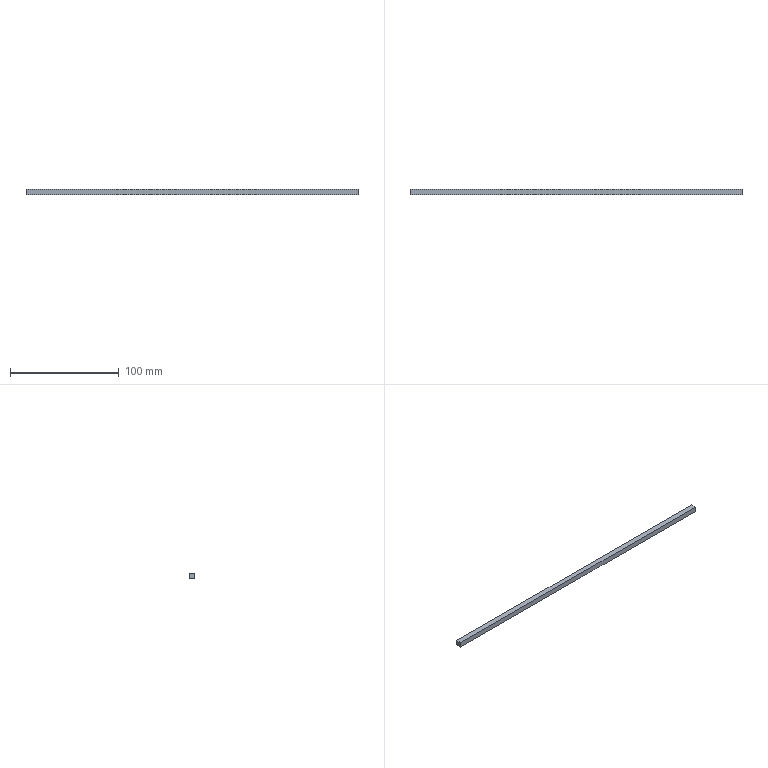Component | SolidWorks | Part23-1 | 1 solid | 6 faces | box 305.58 x 5 x 4.86 mm | volume 7420 mm3 | plane 6
build123d program:
from build123d import *

# Parameters (mm, degrees)
SKETCH1_W           = 4.857
SKETCH1_H           = 5
BOSS_EXTRUDE1_DEPTH = 305.58


with BuildPart() as part:
    # Sketch1 → Boss-Extrude1 (new body)
    with BuildSketch(Plane.XY):
        with Locations((276.879, 308.428)):
            Rectangle(SKETCH1_W, SKETCH1_H)
    extrude(amount=-BOSS_EXTRUDE1_DEPTH)


solid = part.part

# Placed as in the assembly
solid = solid.moved(Location((152.794, -25.683, -135.592), (0, 90, 0)))
STEP:
#1=CARTESIAN_POINT('',(6.016,11.23,-16.143));
#2=VERTEX_POINT('',#1);
#3=CARTESIAN_POINT('',(6.016,11.033,-16.143));
#4=VERTEX_POINT('',#3);
#5=CARTESIAN_POINT('',(6.016,11.23,-16.143));
#6=DIRECTION('',(0.,-1.,0.));
#7=VECTOR('',#6,39.37);
#8=LINE('',#5,#7);
#9=EDGE_CURVE('',#2,#4,#8,.T.);
#10=ORIENTED_EDGE('',*,*,#9,.F.);
#11=CARTESIAN_POINT('',(-6.015,11.23,-16.143));
#12=VERTEX_POINT('',#11);
#13=CARTESIAN_POINT('',(-6.015,11.23,-16.143));
#14=DIRECTION('',(1.,0.,0.));
#15=VECTOR('',#14,39.37);
#16=LINE('',#13,#15);
#17=EDGE_CURVE('',#12,#2,#16,.T.);
#18=ORIENTED_EDGE('',*,*,#17,.F.);
#19=CARTESIAN_POINT('',(-6.015,11.033,-16.143));
#20=VERTEX_POINT('',#19);
#21=CARTESIAN_POINT('',(-6.015,11.23,-16.143));
#22=DIRECTION('',(0.,-1.,0.));
#23=VECTOR('',#22,39.37);
#24=LINE('',#21,#23);
#25=EDGE_CURVE('',#12,#20,#24,.T.);
#26=ORIENTED_EDGE('',*,*,#25,.T.);
#27=CARTESIAN_POINT('',(-6.015,11.033,-16.143));
#28=DIRECTION('',(1.,0.,0.));
#29=VECTOR('',#28,39.37);
#30=LINE('',#27,#29);
#31=EDGE_CURVE('',#20,#4,#30,.T.);
#32=ORIENTED_EDGE('',*,*,#31,.T.);
#33=EDGE_LOOP('',(#10,#18,#26,#32));
#34=FACE_OUTER_BOUND('',#33,.T.);
#35=CARTESIAN_POINT('',(-6.015,11.23,-16.143));
#36=DIRECTION('',(0.,0.,1.));
#37=DIRECTION('',(1.,0.,0.));
#38=AXIS2_PLACEMENT_3D('',#35,#36,#37);
#39=PLANE('',#38);
#40=ADVANCED_FACE('',(#34),#39,.T.);
#41=CARTESIAN_POINT('',(6.016,11.23,-16.335));
#42=VERTEX_POINT('',#41);
#43=CARTESIAN_POINT('',(6.016,11.23,-16.143));
#44=DIRECTION('',(0.,0.,1.));
#45=VECTOR('',#44,39.37);
#46=LINE('',#43,#45);
#47=EDGE_CURVE('',#42,#2,#46,.T.);
#48=ORIENTED_EDGE('',*,*,#47,.F.);
#49=CARTESIAN_POINT('',(-6.015,11.23,-16.335));
#50=VERTEX_POINT('',#49);
#51=CARTESIAN_POINT('',(-6.015,11.23,-16.335));
#52=DIRECTION('',(1.,0.,0.));
#53=VECTOR('',#52,39.37);
#54=LINE('',#51,#53);
#55=EDGE_CURVE('',#50,#42,#54,.T.);
#56=ORIENTED_EDGE('',*,*,#55,.F.);
#57=CARTESIAN_POINT('',(-6.015,11.23,-16.143));
#58=DIRECTION('',(0.,0.,1.));
#59=VECTOR('',#58,39.37);
#60=LINE('',#57,#59);
#61=EDGE_CURVE('',#50,#12,#60,.T.);
#62=ORIENTED_EDGE('',*,*,#61,.T.);
#63=ORIENTED_EDGE('',*,*,#17,.T.);
#64=EDGE_LOOP('',(#48,#56,#62,#63));
#65=FACE_OUTER_BOUND('',#64,.T.);
#66=CARTESIAN_POINT('',(-6.015,11.23,-16.143));
#67=DIRECTION('',(0.,1.,0.));
#68=DIRECTION('',(1.,0.,0.));
#69=AXIS2_PLACEMENT_3D('',#66,#67,#68);
#70=PLANE('',#69);
#71=ADVANCED_FACE('',(#65),#70,.T.);
#72=CARTESIAN_POINT('',(6.016,11.033,-16.335));
#73=VERTEX_POINT('',#72);
#74=CARTESIAN_POINT('',(6.016,11.23,-16.335));
#75=DIRECTION('',(0.,1.,0.));
#76=VECTOR('',#75,39.37);
#77=LINE('',#74,#76);
#78=EDGE_CURVE('',#73,#42,#77,.T.);
#79=ORIENTED_EDGE('',*,*,#78,.F.);
#80=CARTESIAN_POINT('',(-6.015,11.033,-16.335));
#81=VERTEX_POINT('',#80);
#82=CARTESIAN_POINT('',(-6.015,11.033,-16.335));
#83=DIRECTION('',(1.,0.,0.));
#84=VECTOR('',#83,39.37);
#85=LINE('',#82,#84);
#86=EDGE_CURVE('',#81,#73,#85,.T.);
#87=ORIENTED_EDGE('',*,*,#86,.F.);
#88=CARTESIAN_POINT('',(-6.015,11.23,-16.335));
#89=DIRECTION('',(0.,1.,0.));
#90=VECTOR('',#89,39.37);
#91=LINE('',#88,#90);
#92=EDGE_CURVE('',#81,#50,#91,.T.);
#93=ORIENTED_EDGE('',*,*,#92,.T.);
#94=ORIENTED_EDGE('',*,*,#55,.T.);
#95=EDGE_LOOP('',(#79,#87,#93,#94));
#96=FACE_OUTER_BOUND('',#95,.T.);
#97=CARTESIAN_POINT('',(-6.015,11.23,-16.335));
#98=DIRECTION('',(0.,0.,-1.));
#99=DIRECTION('',(-1.,0.,0.));
#100=AXIS2_PLACEMENT_3D('',#97,#98,#99);
#101=PLANE('',#100);
#102=ADVANCED_FACE('',(#96),#101,.T.);
#103=CARTESIAN_POINT('',(6.016,11.033,-16.143));
#104=DIRECTION('',(0.,0.,-1.));
#105=VECTOR('',#104,39.37);
#106=LINE('',#103,#105);
#107=EDGE_CURVE('',#4,#73,#106,.T.);
#108=ORIENTED_EDGE('',*,*,#107,.F.);
#109=ORIENTED_EDGE('',*,*,#31,.F.);
#110=CARTESIAN_POINT('',(-6.015,11.033,-16.143));
#111=DIRECTION('',(0.,0.,-1.));
#112=VECTOR('',#111,39.37);
#113=LINE('',#110,#112);
#114=EDGE_CURVE('',#20,#81,#113,.T.);
#115=ORIENTED_EDGE('',*,*,#114,.T.);
#116=ORIENTED_EDGE('',*,*,#86,.T.);
#117=EDGE_LOOP('',(#108,#109,#115,#116));
#118=FACE_OUTER_BOUND('',#117,.T.);
#119=CARTESIAN_POINT('',(-6.015,11.033,-16.143));
#120=DIRECTION('',(0.,-1.,0.));
#121=DIRECTION('',(-1.,0.,0.));
#122=AXIS2_PLACEMENT_3D('',#119,#120,#121);
#123=PLANE('',#122);
#124=ADVANCED_FACE('',(#118),#123,.T.);
#125=ORIENTED_EDGE('',*,*,#25,.F.);
#126=ORIENTED_EDGE('',*,*,#61,.F.);
#127=ORIENTED_EDGE('',*,*,#92,.F.);
#128=ORIENTED_EDGE('',*,*,#114,.F.);
#129=EDGE_LOOP('',(#125,#126,#127,#128));
#130=FACE_OUTER_BOUND('',#129,.T.);
#131=CARTESIAN_POINT('',(-6.015,-1.011,-5.338));
#132=DIRECTION('',(1.,0.,0.));
#133=DIRECTION('',(0.,0.,-1.));
#134=AXIS2_PLACEMENT_3D('',#131,#132,#133);
#135=PLANE('',#134);
#136=ADVANCED_FACE('',(#130),#135,.F.);
#137=ORIENTED_EDGE('',*,*,#9,.T.);
#138=ORIENTED_EDGE('',*,*,#107,.T.);
#139=ORIENTED_EDGE('',*,*,#78,.T.);
#140=ORIENTED_EDGE('',*,*,#47,.T.);
#141=EDGE_LOOP('',(#137,#138,#139,#140));
#142=FACE_OUTER_BOUND('',#141,.T.);
#143=CARTESIAN_POINT('',(6.016,-1.011,-5.338));
#144=DIRECTION('',(1.,0.,0.));
#145=DIRECTION('',(0.,0.,-1.));
#146=AXIS2_PLACEMENT_3D('',#143,#144,#145);
#147=PLANE('',#146);
#148=ADVANCED_FACE('',(#142),#147,.T.);
#149=CLOSED_SHELL('',(#40,#71,#102,#124,#136,#148));
#150=MANIFOLD_SOLID_BREP('',#149);
#151=CARTESIAN_POINT('',(0.,0.,0.));
#152=DIRECTION('',(0.,0.,1.));
#153=DIRECTION('',(1.,0.,0.));
#154=AXIS2_PLACEMENT_3D('',#151,#152,#153);
#155=(LENGTH_UNIT()NAMED_UNIT(*)SI_UNIT($,.METRE.));
#156=LENGTH_MEASURE_WITH_UNIT(LENGTH_MEASURE(0.0254),#155);
#157=DIMENSIONAL_EXPONENTS(1.,0.,0.,0.,0.,0.,0.);
#158=(CONVERSION_BASED_UNIT('',#156)LENGTH_UNIT()NAMED_UNIT(#157));
#159=UNCERTAINTY_MEASURE_WITH_UNIT(LENGTH_MEASURE(0.00001),#158,'','');
#160=(NAMED_UNIT(*)PLANE_ANGLE_UNIT()SI_UNIT($,.RADIAN.));
#161=(NAMED_UNIT(*)SI_UNIT($,.STERADIAN.)SOLID_ANGLE_UNIT());
#162=(GEOMETRIC_REPRESENTATION_CONTEXT(3)GLOBAL_UNCERTAINTY_ASSIGNED_CONTEXT((#159))GLOBAL_UNIT_ASSIGNED_CONTEXT((#158,#160,#161))REPRESENTATION_CONTEXT('',''));
#163=ADVANCED_BREP_SHAPE_REPRESENTATION('',(#150,#154),#162);
#164=COLOUR_RGB('',0.7922,0.8196,0.9333);
#165=FILL_AREA_STYLE_COLOUR('',#164);
#166=FILL_AREA_STYLE('',(#165));
#167=SURFACE_STYLE_FILL_AREA(#166);
#168=SURFACE_SIDE_STYLE('',(#167));
#169=SURFACE_STYLE_USAGE(.BOTH.,#168);
#170=PRESENTATION_STYLE_ASSIGNMENT((#169));
#171=STYLED_ITEM('',(#170),#150);
#172=(LENGTH_UNIT()NAMED_UNIT(*)SI_UNIT($,.METRE.));
#173=LENGTH_MEASURE_WITH_UNIT(LENGTH_MEASURE(0.0254),#172);
#174=DIMENSIONAL_EXPONENTS(1.,0.,0.,0.,0.,0.,0.);
#175=(CONVERSION_BASED_UNIT('',#173)LENGTH_UNIT()NAMED_UNIT(#174));
#176=UNCERTAINTY_MEASURE_WITH_UNIT(LENGTH_MEASURE(0.00001),#175,'','');
#177=(NAMED_UNIT(*)PLANE_ANGLE_UNIT()SI_UNIT($,.RADIAN.));
#178=(NAMED_UNIT(*)SI_UNIT($,.STERADIAN.)SOLID_ANGLE_UNIT());
#179=(GEOMETRIC_REPRESENTATION_CONTEXT(3)GLOBAL_UNCERTAINTY_ASSIGNED_CONTEXT((#176))GLOBAL_UNIT_ASSIGNED_CONTEXT((#175,#177,#178))REPRESENTATION_CONTEXT('',''));
#180=MECHANICAL_DESIGN_GEOMETRIC_PRESENTATION_REPRESENTATION('',(#171),#179);
#181=PRESENTATION_LAYER_ASSIGNMENT('','',(#171));